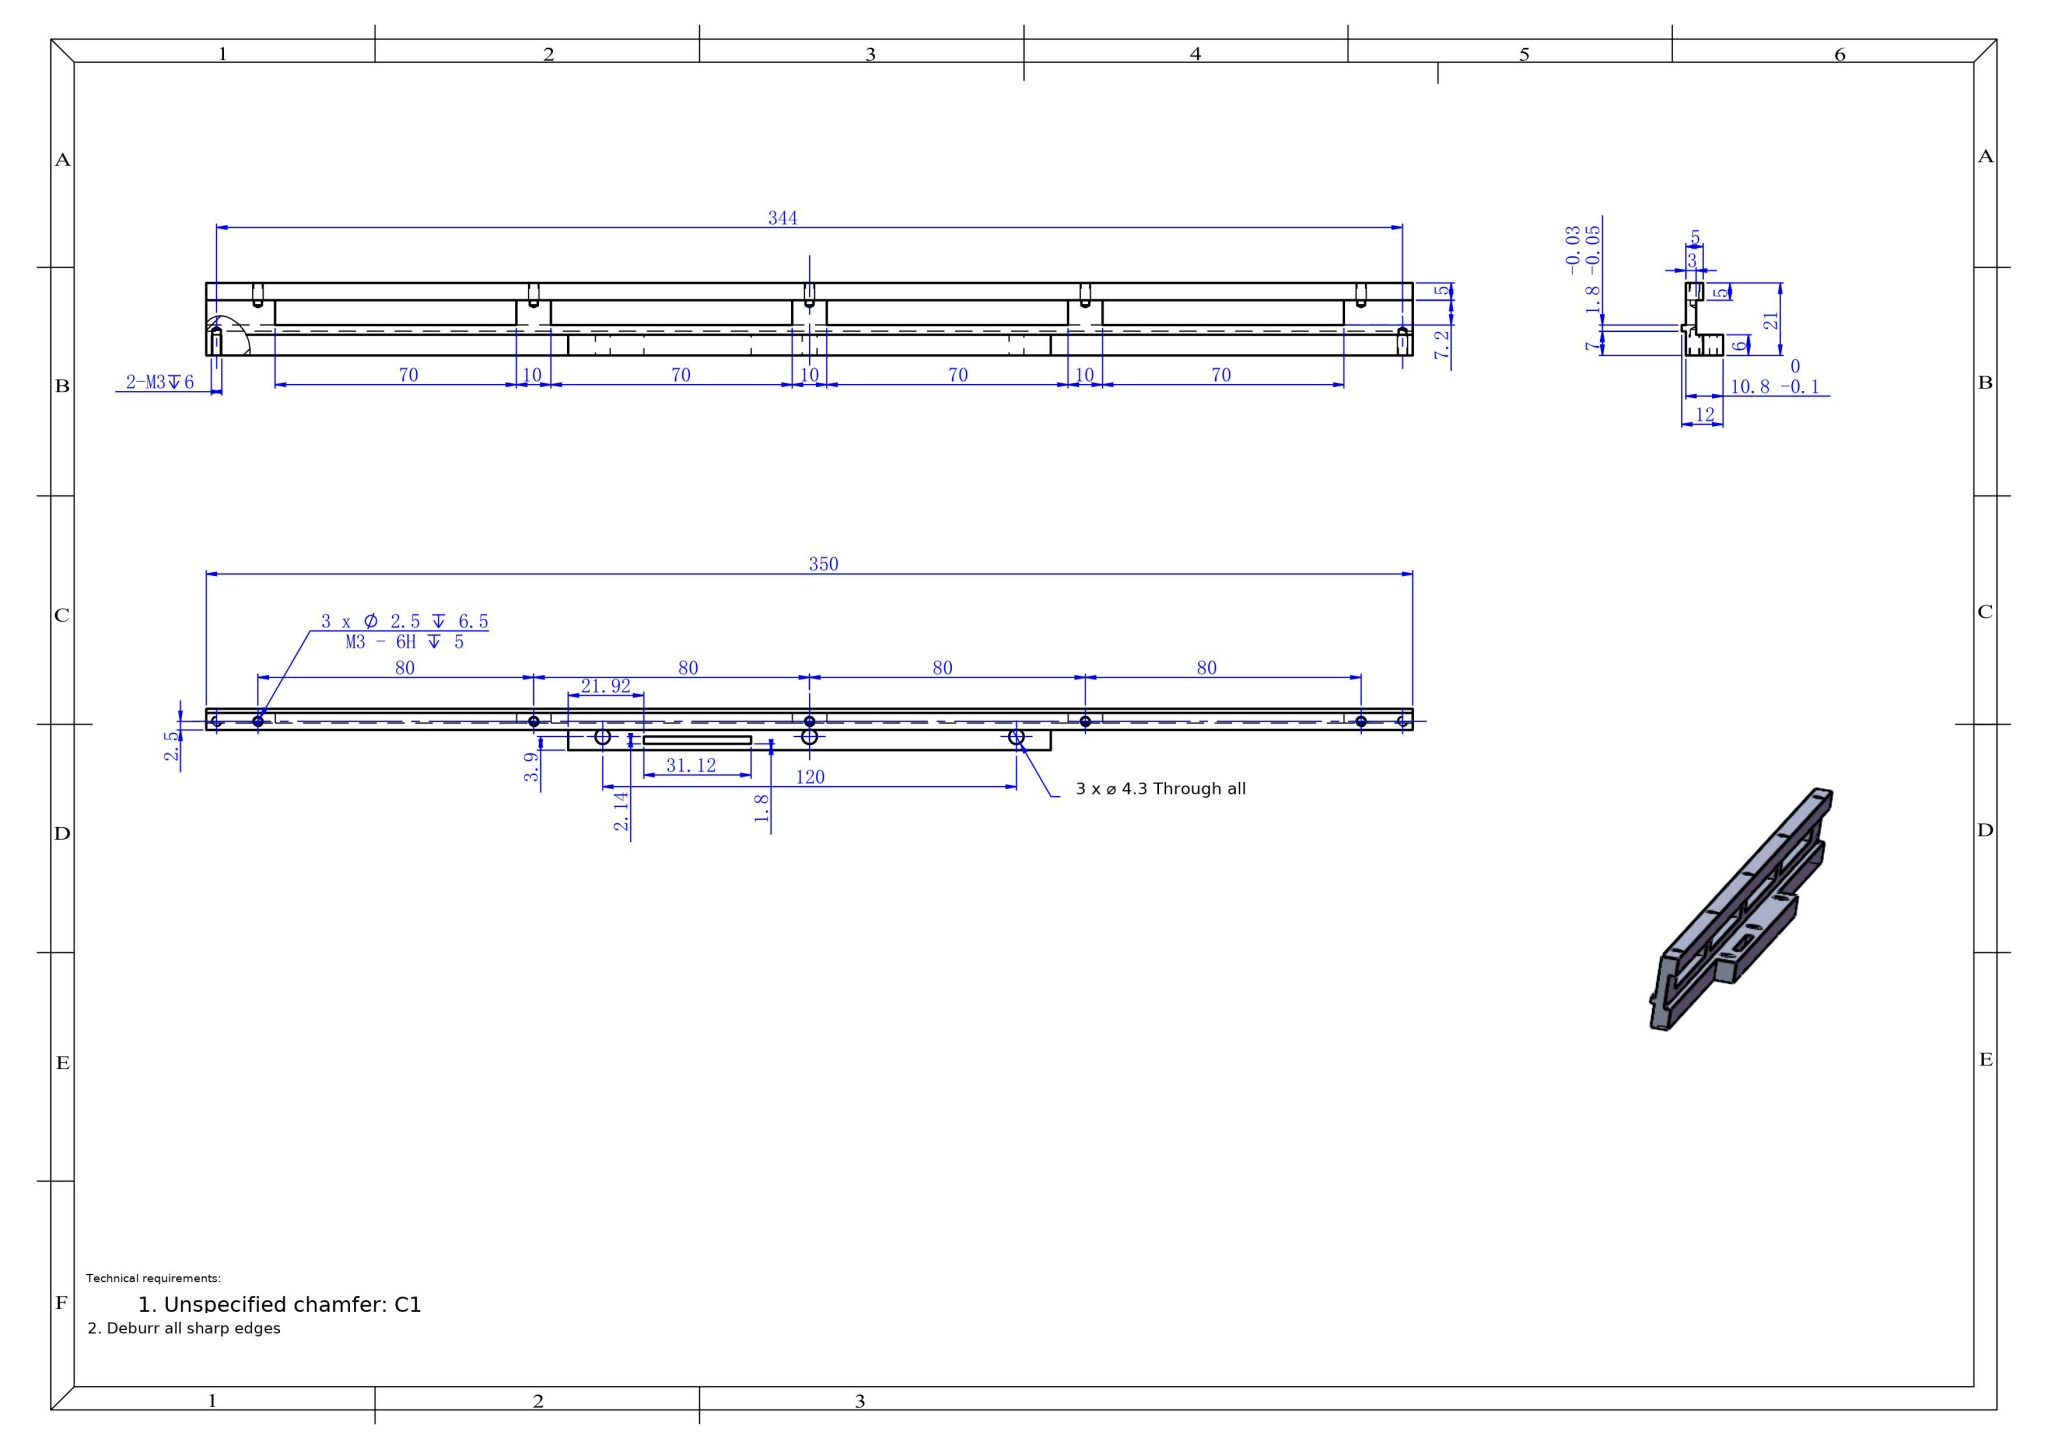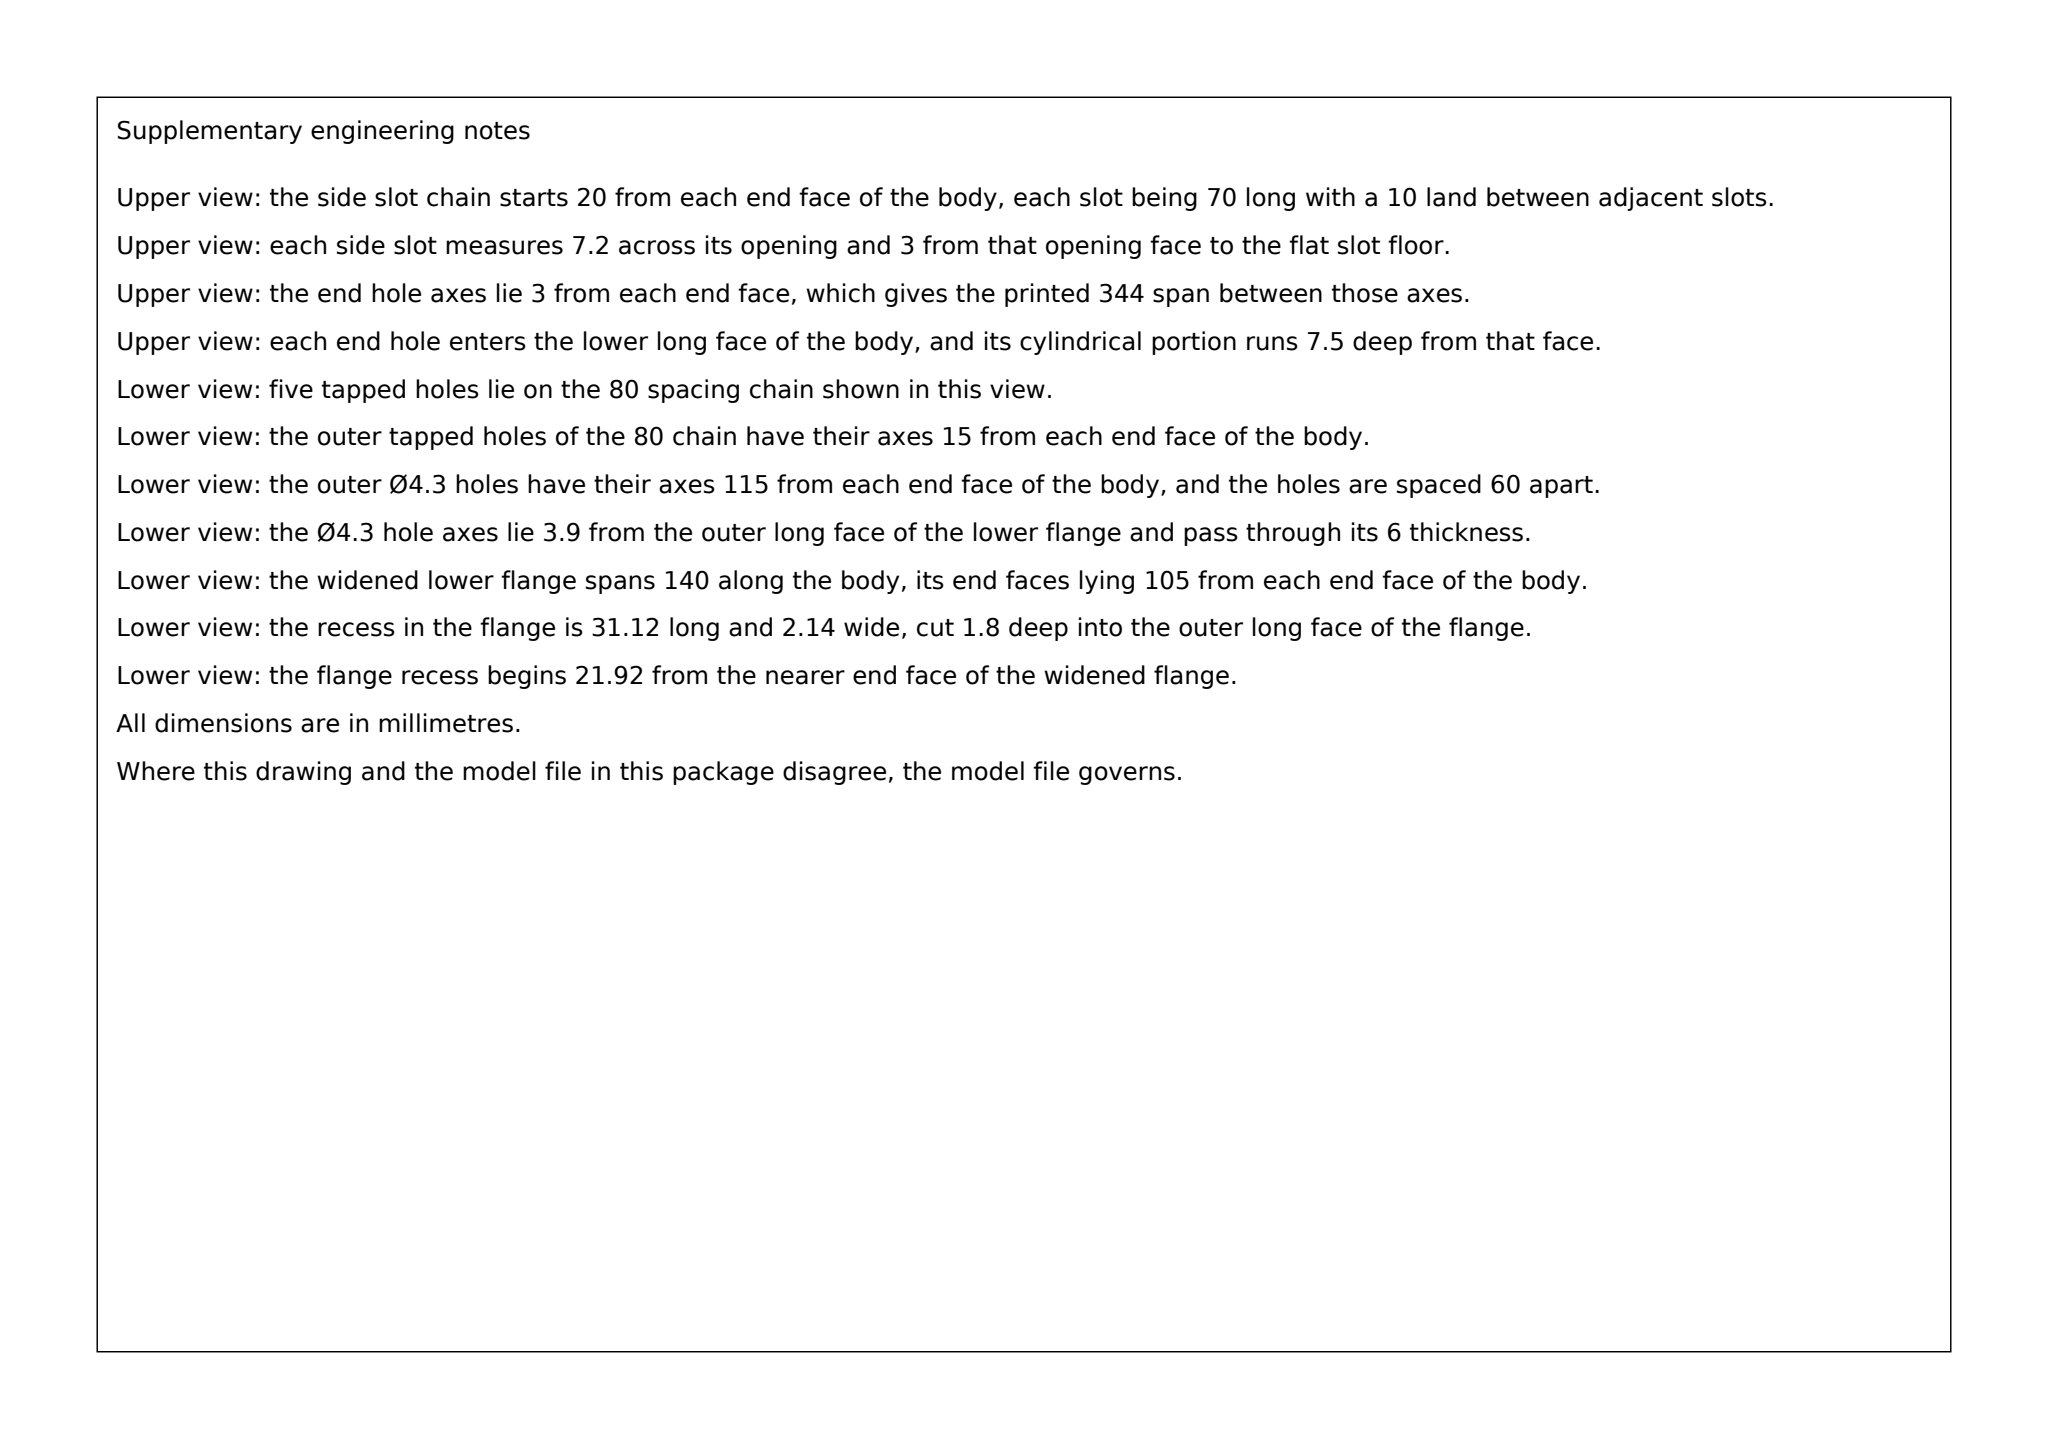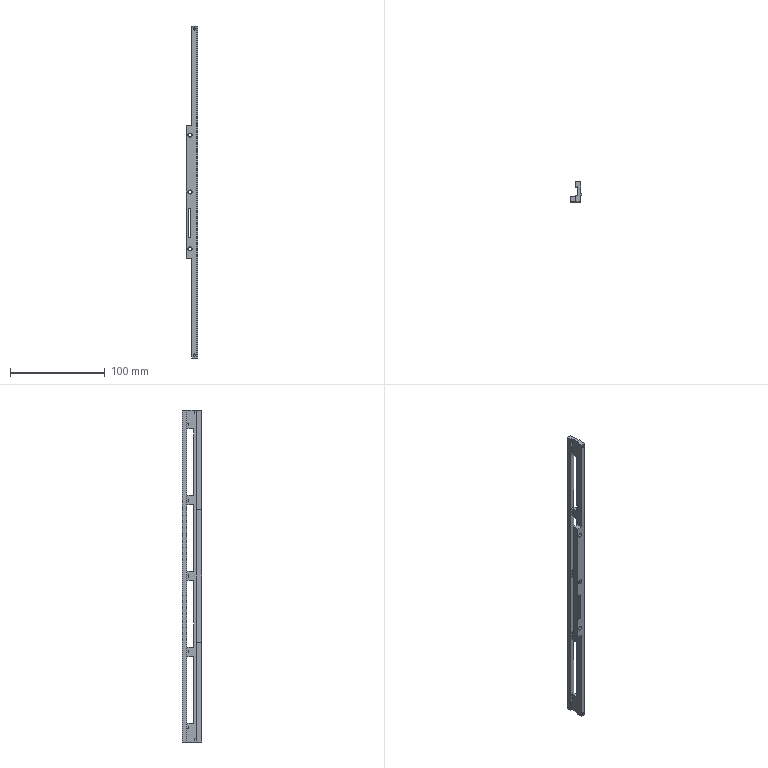Part | SolidWorks | mm | 1 solid | 64 faces | box 12 x 21 x 350 mm | volume 28442 mm3 | plane 30 | cylinder 20 | cone 14 | commonest cylinder face diameters 2.5 x14 4.3 x6
Drawing notes:
OVERALL 12 W X 21 H X 350 LG | from the solid: bbox_xyz 12.001 x 21.001 x 350.001
RIB 2 THK, 5.8-7.8 FROM BACK FACE; WALL 1.8; BASE 6 THK | from the solid: x planes 0/1.8/3.94/5.8/7.8/10.8/12.0; y planes 0/6/7/8.8/16/21
2 X M3 DP 6 (DRILL Ø2.5 DP 7.5) AT 3 & 347 FROM LH END, 8.3 FROM BACK | from the solid: Ø2.5 y-axis holes at z=3.0 and z=347.0, x=8.3, length 7.5
5 X Ø2.5 DP 6.5 / M3-6H DP 5 AT 15,95,175,255,335 FROM LH END, 8.3 FROM BACK | from the solid: Ø2.5 y-axis holes len 6.5 at z=15/95/175/255/335, x=8.3
3 X Ø4.3 THRU AT 115, 175, 235 FROM LH END, 3.9 FROM BACK FACE | from the solid: Ø4.3 y-axis holes at z=115/175/235, x=3.9, length 6.0
DRILL PT 118° TYP ALL Ø2.5 HOLES | from the solid: cones [118.0, ref_dia 2.5, 14]
SLOT 31.12 LG X 1.8 W X 2.14 DP, SQ ENDS, STARTS 126.92 FROM LH END | from the solid: z planes 126.92 & 158.04 (31.12 lg); x planes 1.8 & 3.94 (2.14 dp)
build123d program:
from build123d import *

# Parameters (mm, degrees)
SKETCH1_W                      = 12
SKETCH1_H                      = 21
BOSS_EXTRUDE1_DEPTH            = 350
SKETCH2_W                      = 1.2
SKETCH2_H                      = 12.2
SKETCH2_H_2                    = 7
CUT_EXTRUDE1_DEPTH             = 358.917
SKETCH3_W                      = 5.8
SKETCH3_H                      = 15
CUT_EXTRUDE2_DEPTH             = 358.917
M3_TAPPED_HOLE1_AT_2_COUNT     = 2
M3_TAPPED_HOLE1_AT_2_PITCH     = 80
M3_TAPPED_HOLE1_AT_3_COUNT     = 2
M3_TAPPED_HOLE1_AT_3_PITCH     = 80
SKETCH6_W                      = 70
SKETCH6_H                      = 7.2
CUT_EXTRUDE3_DEPTH             = 355.932
SKETCH7_W                      = 2
SKETCH7_H                      = 10
CUT_EXTRUDE4_DEPTH             = 358.917
SKETCH8_W                      = 5.8
SKETCH8_H                      = 105
CUT_EXTRUDE5_DEPTH             = 354.4
F_4_3_4_3_DIAMETER_HOLE1_D     = 4.3
F_4_3_4_3_DIAMETER_HOLE1_DEPTH = 6
SKETCH13_W                     = 2.136
SKETCH13_H                     = 31.119
CUT_EXTRUDE6_DEPTH             = 29


with BuildPart() as part:
    # Sketch1 → Boss-Extrude1 (new body)
    with BuildSketch(Plane.XY):
        with Locations((-40.543, 48.139)):
            Rectangle(SKETCH1_W, SKETCH1_H)
    extrude(amount=BOSS_EXTRUDE1_DEPTH)

    # Sketch2 → Cut-Extrude1 (cut, through all)
    with BuildSketch(Plane.XY.offset(350)):
        with Locations((-35.143, 52.539)):
            Rectangle(SKETCH2_W, SKETCH2_H)
        with Locations((-35.143, 41.139)):
            Rectangle(SKETCH2_W, SKETCH2_H_2)
    extrude(amount=-CUT_EXTRUDE1_DEPTH, mode=Mode.SUBTRACT)

    # Sketch3 → Cut-Extrude2 (cut, through all)
    with BuildSketch(Plane.XY.offset(350)):
        with Locations((-43.643, 51.139)):
            Rectangle(SKETCH3_W, SKETCH3_H)
    extrude(amount=-CUT_EXTRUDE2_DEPTH, mode=Mode.SUBTRACT)

    # Sketch5 → M3 Tapped Hole1 (revolve, cut)
    with BuildSketch(Plane(origin=(-38.243, 58.639, 95), x_dir=(0, 0, 1), z_dir=(1, 0, 0))):
        Polygon((0, 0), (0, 7.251), (1.25, 6.5), (1.25, 0), align=None)
    m3_tapped_hole1 = revolve(axis=Axis((-38.243, 64.989, 95), (0, -1, 0)), mode=Mode.SUBTRACT)

    # M3 Tapped Hole1 at 2: M3 Tapped Hole1 ×2
    with Locations(*[(0, 0, i * M3_TAPPED_HOLE1_AT_2_PITCH) for i in range(1, M3_TAPPED_HOLE1_AT_2_COUNT)]):
        add(m3_tapped_hole1, mode=Mode.SUBTRACT)

    # M3 Tapped Hole1 at 3: M3 Tapped Hole1 ×2
    with Locations(*[(0, 0, -i * M3_TAPPED_HOLE1_AT_3_PITCH) for i in range(1, M3_TAPPED_HOLE1_AT_3_COUNT)]):
        add(m3_tapped_hole1, mode=Mode.SUBTRACT)

    # Mirror1: M3 Tapped Hole1 across plane
    add(m3_tapped_hole1.mirror(Plane.XY.offset(175)), mode=Mode.SUBTRACT)

    # Mirror1 copy 1 sketch → Mirror1 copy 1 (revolve, cut)
    with BuildSketch(Plane(origin=(-38.243, 58.639, 175), x_dir=(0, 0, -1), z_dir=(1, 0, 0))):
        Polygon((0, 0), (0, -7.251), (1.25, -6.5), (1.25, 0), align=None)
    revolve(axis=Axis((-38.243, 64.989, 175), (0, 1, 0)), mode=Mode.SUBTRACT)

    # Mirror1 copy 2 sketch → Mirror1 copy 2 (revolve, cut)
    with BuildSketch(Plane(origin=(-38.243, 58.639, 335), x_dir=(0, 0, -1), z_dir=(1, 0, 0))):
        Polygon((0, 0), (0, -7.251), (1.25, -6.5), (1.25, 0), align=None)
    revolve(axis=Axis((-38.243, 64.989, 335), (0, 1, 0)), mode=Mode.SUBTRACT)

    # Sketch6 → Cut-Extrude3 (cut, through all)
    with BuildSketch(Plane.ZY.offset(40.743)):
        with Locations((55, 50.039)):
            Rectangle(SKETCH6_W, SKETCH6_H)
        with Locations((135, 50.039)):
            Rectangle(SKETCH6_W, SKETCH6_H)
        with Locations((215, 50.039)):
            Rectangle(SKETCH6_W, SKETCH6_H)
        with Locations((295, 50.039)):
            Rectangle(SKETCH6_W, SKETCH6_H)
    extrude(amount=-CUT_EXTRUDE3_DEPTH, mode=Mode.SUBTRACT)

    # Sketch7 → Cut-Extrude4 (cut, through all)
    with BuildSketch(Plane.XY.offset(350)):
        with Locations((-39.743, 48.639)):
            Rectangle(SKETCH7_W, SKETCH7_H)
    extrude(amount=-CUT_EXTRUDE4_DEPTH, mode=Mode.SUBTRACT)

    # Sketch8 → Cut-Extrude5 (cut, through all)
    with BuildSketch(Plane(origin=(0, 43.639, 0), x_dir=(1, 0, 0), z_dir=(0, 1, 0))):
        with Locations((-43.643, -52.5)):
            Rectangle(SKETCH8_W, SKETCH8_H)
        with Locations((-43.643, -297.5)):
            Rectangle(SKETCH8_W, SKETCH8_H)
    extrude(amount=-CUT_EXTRUDE5_DEPTH, mode=Mode.SUBTRACT)

    # 4.3 _4.3_ Diameter Hole1
    with Locations(Plane(origin=(0, 43.639, 0), x_dir=(1, 0, 0), z_dir=(0, 1, 0))):
        with Locations((-42.643, -115), (-42.643, -175), (-42.643, -235)):
            Hole(F_4_3_4_3_DIAMETER_HOLE1_D / 2, depth=F_4_3_4_3_DIAMETER_HOLE1_DEPTH)

    # Sketch12 → M3 Tapped Hole2 (revolve, cut)
    with BuildSketch(Plane(origin=(-38.243, 37.639, 347), x_dir=(0, 0, -1), z_dir=(1, 0, 0))):
        Polygon((0, 0), (0, 8.251), (1.25, 7.5), (1.25, 0), align=None)
    m3_tapped_hole2 = revolve(axis=Axis((-38.243, 31.289, 347), (0, 1, 0)), mode=Mode.SUBTRACT)

    # Mirror2: M3 Tapped Hole2 across plane
    add(m3_tapped_hole2.mirror(Plane.XY.offset(175)), mode=Mode.SUBTRACT)

    # Sketch13 → Cut-Extrude6 (cut)
    with BuildSketch(Plane(origin=(0, 43.639, 0), x_dir=(1, 0, 0), z_dir=(0, 1, 0))):
        with Locations((-43.673, -142.483)):
            Rectangle(SKETCH13_W, SKETCH13_H)
    extrude(amount=-CUT_EXTRUDE6_DEPTH, mode=Mode.SUBTRACT)


solid = part.part